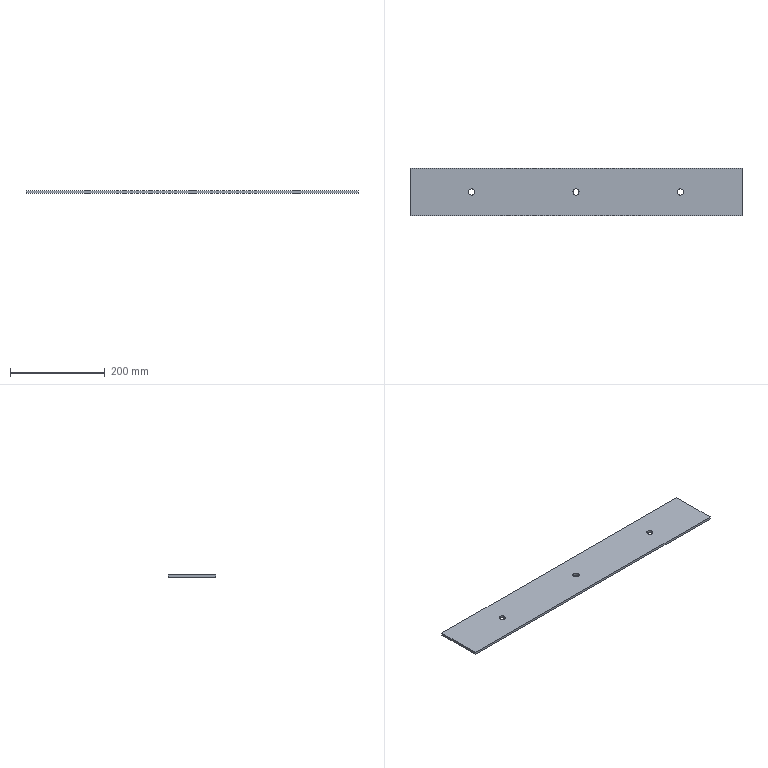Component | NX | SIDE_CONN_PLATE | 1 solid | 9 faces | box 700 x 100 x 5 mm | volume 348009 mm3 | plane 6 | cylinder 3 | commonest cylinder face diameters 13 x3
STEP:
#1=CARTESIAN_POINT('',(0.,0.,0.));
#2=DIRECTION('',(0.,0.,1.));
#3=DIRECTION('',(1.,0.,0.));
#4=AXIS2_PLACEMENT_3D('',#1,#2,#3);
#5=CARTESIAN_POINT('',(650.,50.,-525.));
#6=VERTEX_POINT('',#5);
#7=CARTESIAN_POINT('',(-50.,50.,-525.));
#8=VERTEX_POINT('',#7);
#9=CARTESIAN_POINT('',(650.,50.,-525.));
#10=DIRECTION('',(-1.,0.,0.));
#11=VECTOR('',#10,1.);
#12=LINE('',#9,#11);
#13=CARTESIAN_POINT('',(650.,50.,-530.));
#14=DIRECTION('',(0.,1.,0.));
#15=DIRECTION('',(0.,0.,1.));
#16=AXIS2_PLACEMENT_3D('',#13,#14,#15);
#17=PLANE('',#16);
#18=CARTESIAN_POINT('',(5.,0.));
#19=DIRECTION('',(0.,-1.));
#20=VECTOR('',#19,1.);
#21=LINE('',#18,#20);
#22=(GEOMETRIC_REPRESENTATION_CONTEXT(2)PARAMETRIC_REPRESENTATION_CONTEXT()REPRESENTATION_CONTEXT('',''));
#23=DEFINITIONAL_REPRESENTATION('',(#21),#22);
#24=PCURVE('',#17,#23);
#25=CARTESIAN_POINT('',(520.,-0.,-525.));
#26=DIRECTION('',(0.,0.,-1.));
#27=DIRECTION('',(1.,0.,0.));
#28=AXIS2_PLACEMENT_3D('',#25,#26,#27);
#29=PLANE('',#28);
#30=CARTESIAN_POINT('',(130.,-50.));
#31=DIRECTION('',(-1.,0.));
#32=VECTOR('',#31,1.);
#33=LINE('',#30,#32);
#34=(GEOMETRIC_REPRESENTATION_CONTEXT(2)PARAMETRIC_REPRESENTATION_CONTEXT()REPRESENTATION_CONTEXT('',''));
#35=DEFINITIONAL_REPRESENTATION('',(#33),#34);
#36=PCURVE('',#29,#35);
#37=SURFACE_CURVE('',#12,(#24,#36),.PCURVE_S1.);
#38=EDGE_CURVE('',#6,#8,#37,.T.);
#39=ORIENTED_EDGE('',*,*,#38,.F.);
#40=CARTESIAN_POINT('',(650.,50.,-530.));
#41=VERTEX_POINT('',#40);
#42=CARTESIAN_POINT('',(650.,50.,-530.));
#43=DIRECTION('',(0.,0.,1.));
#44=VECTOR('',#43,1.);
#45=LINE('',#42,#44);
#46=CARTESIAN_POINT('',(0.,0.));
#47=DIRECTION('',(1.,0.));
#48=VECTOR('',#47,1.);
#49=LINE('',#46,#48);
#50=(GEOMETRIC_REPRESENTATION_CONTEXT(2)PARAMETRIC_REPRESENTATION_CONTEXT()REPRESENTATION_CONTEXT('',''));
#51=DEFINITIONAL_REPRESENTATION('',(#49),#50);
#52=PCURVE('',#17,#51);
#53=CARTESIAN_POINT('',(650.,-50.,-530.));
#54=DIRECTION('',(1.,0.,0.));
#55=DIRECTION('',(0.,0.,1.));
#56=AXIS2_PLACEMENT_3D('',#53,#54,#55);
#57=PLANE('',#56);
#58=CARTESIAN_POINT('',(0.,-100.));
#59=DIRECTION('',(1.,0.));
#60=VECTOR('',#59,1.);
#61=LINE('',#58,#60);
#62=(GEOMETRIC_REPRESENTATION_CONTEXT(2)PARAMETRIC_REPRESENTATION_CONTEXT()REPRESENTATION_CONTEXT('',''));
#63=DEFINITIONAL_REPRESENTATION('',(#61),#62);
#64=PCURVE('',#57,#63);
#65=SURFACE_CURVE('',#45,(#52,#64),.PCURVE_S1.);
#66=EDGE_CURVE('',#41,#6,#65,.T.);
#67=ORIENTED_EDGE('',*,*,#66,.F.);
#68=CARTESIAN_POINT('',(-50.,50.,-530.));
#69=VERTEX_POINT('',#68);
#70=CARTESIAN_POINT('',(650.,50.,-530.));
#71=DIRECTION('',(-1.,0.,0.));
#72=VECTOR('',#71,1.);
#73=LINE('',#70,#72);
#74=CARTESIAN_POINT('',(0.,0.));
#75=DIRECTION('',(0.,-1.));
#76=VECTOR('',#75,1.);
#77=LINE('',#74,#76);
#78=(GEOMETRIC_REPRESENTATION_CONTEXT(2)PARAMETRIC_REPRESENTATION_CONTEXT()REPRESENTATION_CONTEXT('',''));
#79=DEFINITIONAL_REPRESENTATION('',(#77),#78);
#80=PCURVE('',#17,#79);
#81=CARTESIAN_POINT('',(520.,-0.,-530.));
#82=DIRECTION('',(0.,0.,-1.));
#83=DIRECTION('',(1.,0.,0.));
#84=AXIS2_PLACEMENT_3D('',#81,#82,#83);
#85=PLANE('',#84);
#86=CARTESIAN_POINT('',(130.,-50.));
#87=DIRECTION('',(-1.,0.));
#88=VECTOR('',#87,1.);
#89=LINE('',#86,#88);
#90=(GEOMETRIC_REPRESENTATION_CONTEXT(2)PARAMETRIC_REPRESENTATION_CONTEXT()REPRESENTATION_CONTEXT('',''));
#91=DEFINITIONAL_REPRESENTATION('',(#89),#90);
#92=PCURVE('',#85,#91);
#93=SURFACE_CURVE('',#73,(#80,#92),.PCURVE_S1.);
#94=EDGE_CURVE('',#41,#69,#93,.T.);
#95=ORIENTED_EDGE('',*,*,#94,.T.);
#96=CARTESIAN_POINT('',(-50.,50.,-530.));
#97=DIRECTION('',(0.,0.,1.));
#98=VECTOR('',#97,1.);
#99=LINE('',#96,#98);
#100=CARTESIAN_POINT('',(0.,-700.));
#101=DIRECTION('',(1.,0.));
#102=VECTOR('',#101,1.);
#103=LINE('',#100,#102);
#104=(GEOMETRIC_REPRESENTATION_CONTEXT(2)PARAMETRIC_REPRESENTATION_CONTEXT()REPRESENTATION_CONTEXT('',''));
#105=DEFINITIONAL_REPRESENTATION('',(#103),#104);
#106=PCURVE('',#17,#105);
#107=CARTESIAN_POINT('',(-50.,50.,-530.));
#108=DIRECTION('',(-1.,0.,0.));
#109=DIRECTION('',(0.,0.,-1.));
#110=AXIS2_PLACEMENT_3D('',#107,#108,#109);
#111=PLANE('',#110);
#112=CARTESIAN_POINT('',(0.,0.));
#113=DIRECTION('',(-1.,0.));
#114=VECTOR('',#113,1.);
#115=LINE('',#112,#114);
#116=(GEOMETRIC_REPRESENTATION_CONTEXT(2)PARAMETRIC_REPRESENTATION_CONTEXT()REPRESENTATION_CONTEXT('',''));
#117=DEFINITIONAL_REPRESENTATION('',(#115),#116);
#118=PCURVE('',#111,#117);
#119=SURFACE_CURVE('',#99,(#106,#118),.PCURVE_S1.);
#120=EDGE_CURVE('',#69,#8,#119,.T.);
#121=ORIENTED_EDGE('',*,*,#120,.T.);
#122=EDGE_LOOP('',(#39,#67,#95,#121));
#123=FACE_BOUND('',#122,.T.);
#124=ADVANCED_FACE('',(#123),#17,.T.);
#125=CARTESIAN_POINT('',(-50.,-50.,-525.));
#126=VERTEX_POINT('',#125);
#127=CARTESIAN_POINT('',(-50.,50.,-525.));
#128=DIRECTION('',(0.,-1.,0.));
#129=VECTOR('',#128,1.);
#130=LINE('',#127,#129);
#131=CARTESIAN_POINT('',(-5.,0.));
#132=DIRECTION('',(0.,1.));
#133=VECTOR('',#132,1.);
#134=LINE('',#131,#133);
#135=(GEOMETRIC_REPRESENTATION_CONTEXT(2)PARAMETRIC_REPRESENTATION_CONTEXT()REPRESENTATION_CONTEXT('',''));
#136=DEFINITIONAL_REPRESENTATION('',(#134),#135);
#137=PCURVE('',#111,#136);
#138=CARTESIAN_POINT('',(-570.,-50.));
#139=DIRECTION('',(0.,1.));
#140=VECTOR('',#139,1.);
#141=LINE('',#138,#140);
#142=(GEOMETRIC_REPRESENTATION_CONTEXT(2)PARAMETRIC_REPRESENTATION_CONTEXT()REPRESENTATION_CONTEXT('',''));
#143=DEFINITIONAL_REPRESENTATION('',(#141),#142);
#144=PCURVE('',#29,#143);
#145=SURFACE_CURVE('',#130,(#137,#144),.PCURVE_S1.);
#146=EDGE_CURVE('',#8,#126,#145,.T.);
#147=ORIENTED_EDGE('',*,*,#146,.F.);
#148=ORIENTED_EDGE('',*,*,#120,.F.);
#149=CARTESIAN_POINT('',(-50.,-50.,-530.));
#150=VERTEX_POINT('',#149);
#151=CARTESIAN_POINT('',(-50.,50.,-530.));
#152=DIRECTION('',(0.,-1.,0.));
#153=VECTOR('',#152,1.);
#154=LINE('',#151,#153);
#155=CARTESIAN_POINT('',(0.,0.));
#156=DIRECTION('',(0.,1.));
#157=VECTOR('',#156,1.);
#158=LINE('',#155,#157);
#159=(GEOMETRIC_REPRESENTATION_CONTEXT(2)PARAMETRIC_REPRESENTATION_CONTEXT()REPRESENTATION_CONTEXT('',''));
#160=DEFINITIONAL_REPRESENTATION('',(#158),#159);
#161=PCURVE('',#111,#160);
#162=CARTESIAN_POINT('',(-570.,-50.));
#163=DIRECTION('',(0.,1.));
#164=VECTOR('',#163,1.);
#165=LINE('',#162,#164);
#166=(GEOMETRIC_REPRESENTATION_CONTEXT(2)PARAMETRIC_REPRESENTATION_CONTEXT()REPRESENTATION_CONTEXT('',''));
#167=DEFINITIONAL_REPRESENTATION('',(#165),#166);
#168=PCURVE('',#85,#167);
#169=SURFACE_CURVE('',#154,(#161,#168),.PCURVE_S1.);
#170=EDGE_CURVE('',#69,#150,#169,.T.);
#171=ORIENTED_EDGE('',*,*,#170,.T.);
#172=CARTESIAN_POINT('',(-50.,-50.,-530.));
#173=DIRECTION('',(0.,0.,1.));
#174=VECTOR('',#173,1.);
#175=LINE('',#172,#174);
#176=CARTESIAN_POINT('',(0.,100.));
#177=DIRECTION('',(-1.,0.));
#178=VECTOR('',#177,1.);
#179=LINE('',#176,#178);
#180=(GEOMETRIC_REPRESENTATION_CONTEXT(2)PARAMETRIC_REPRESENTATION_CONTEXT()REPRESENTATION_CONTEXT('',''));
#181=DEFINITIONAL_REPRESENTATION('',(#179),#180);
#182=PCURVE('',#111,#181);
#183=CARTESIAN_POINT('',(-50.,-50.,-530.));
#184=DIRECTION('',(0.,-1.,0.));
#185=DIRECTION('',(0.,0.,-1.));
#186=AXIS2_PLACEMENT_3D('',#183,#184,#185);
#187=PLANE('',#186);
#188=CARTESIAN_POINT('',(0.,0.));
#189=DIRECTION('',(-1.,0.));
#190=VECTOR('',#189,1.);
#191=LINE('',#188,#190);
#192=(GEOMETRIC_REPRESENTATION_CONTEXT(2)PARAMETRIC_REPRESENTATION_CONTEXT()REPRESENTATION_CONTEXT('',''));
#193=DEFINITIONAL_REPRESENTATION('',(#191),#192);
#194=PCURVE('',#187,#193);
#195=SURFACE_CURVE('',#175,(#182,#194),.PCURVE_S1.);
#196=EDGE_CURVE('',#150,#126,#195,.T.);
#197=ORIENTED_EDGE('',*,*,#196,.T.);
#198=EDGE_LOOP('',(#147,#148,#171,#197));
#199=FACE_BOUND('',#198,.T.);
#200=ADVANCED_FACE('',(#199),#111,.T.);
#201=CARTESIAN_POINT('',(650.,-50.,-525.));
#202=VERTEX_POINT('',#201);
#203=CARTESIAN_POINT('',(-50.,-50.,-525.));
#204=DIRECTION('',(1.,0.,0.));
#205=VECTOR('',#204,1.);
#206=LINE('',#203,#205);
#207=CARTESIAN_POINT('',(-5.,0.));
#208=DIRECTION('',(0.,1.));
#209=VECTOR('',#208,1.);
#210=LINE('',#207,#209);
#211=(GEOMETRIC_REPRESENTATION_CONTEXT(2)PARAMETRIC_REPRESENTATION_CONTEXT()REPRESENTATION_CONTEXT('',''));
#212=DEFINITIONAL_REPRESENTATION('',(#210),#211);
#213=PCURVE('',#187,#212);
#214=CARTESIAN_POINT('',(-570.,50.));
#215=DIRECTION('',(1.,0.));
#216=VECTOR('',#215,1.);
#217=LINE('',#214,#216);
#218=(GEOMETRIC_REPRESENTATION_CONTEXT(2)PARAMETRIC_REPRESENTATION_CONTEXT()REPRESENTATION_CONTEXT('',''));
#219=DEFINITIONAL_REPRESENTATION('',(#217),#218);
#220=PCURVE('',#29,#219);
#221=SURFACE_CURVE('',#206,(#213,#220),.PCURVE_S1.);
#222=EDGE_CURVE('',#126,#202,#221,.T.);
#223=ORIENTED_EDGE('',*,*,#222,.F.);
#224=ORIENTED_EDGE('',*,*,#196,.F.);
#225=CARTESIAN_POINT('',(650.,-50.,-530.));
#226=VERTEX_POINT('',#225);
#227=CARTESIAN_POINT('',(-50.,-50.,-530.));
#228=DIRECTION('',(1.,0.,0.));
#229=VECTOR('',#228,1.);
#230=LINE('',#227,#229);
#231=CARTESIAN_POINT('',(0.,0.));
#232=DIRECTION('',(0.,1.));
#233=VECTOR('',#232,1.);
#234=LINE('',#231,#233);
#235=(GEOMETRIC_REPRESENTATION_CONTEXT(2)PARAMETRIC_REPRESENTATION_CONTEXT()REPRESENTATION_CONTEXT('',''));
#236=DEFINITIONAL_REPRESENTATION('',(#234),#235);
#237=PCURVE('',#187,#236);
#238=CARTESIAN_POINT('',(-570.,50.));
#239=DIRECTION('',(1.,0.));
#240=VECTOR('',#239,1.);
#241=LINE('',#238,#240);
#242=(GEOMETRIC_REPRESENTATION_CONTEXT(2)PARAMETRIC_REPRESENTATION_CONTEXT()REPRESENTATION_CONTEXT('',''));
#243=DEFINITIONAL_REPRESENTATION('',(#241),#242);
#244=PCURVE('',#85,#243);
#245=SURFACE_CURVE('',#230,(#237,#244),.PCURVE_S1.);
#246=EDGE_CURVE('',#150,#226,#245,.T.);
#247=ORIENTED_EDGE('',*,*,#246,.T.);
#248=CARTESIAN_POINT('',(650.,-50.,-530.));
#249=DIRECTION('',(0.,0.,1.));
#250=VECTOR('',#249,1.);
#251=LINE('',#248,#250);
#252=CARTESIAN_POINT('',(0.,700.));
#253=DIRECTION('',(-1.,0.));
#254=VECTOR('',#253,1.);
#255=LINE('',#252,#254);
#256=(GEOMETRIC_REPRESENTATION_CONTEXT(2)PARAMETRIC_REPRESENTATION_CONTEXT()REPRESENTATION_CONTEXT('',''));
#257=DEFINITIONAL_REPRESENTATION('',(#255),#256);
#258=PCURVE('',#187,#257);
#259=CARTESIAN_POINT('',(0.,0.));
#260=DIRECTION('',(1.,0.));
#261=VECTOR('',#260,1.);
#262=LINE('',#259,#261);
#263=(GEOMETRIC_REPRESENTATION_CONTEXT(2)PARAMETRIC_REPRESENTATION_CONTEXT()REPRESENTATION_CONTEXT('',''));
#264=DEFINITIONAL_REPRESENTATION('',(#262),#263);
#265=PCURVE('',#57,#264);
#266=SURFACE_CURVE('',#251,(#258,#265),.PCURVE_S1.);
#267=EDGE_CURVE('',#226,#202,#266,.T.);
#268=ORIENTED_EDGE('',*,*,#267,.T.);
#269=EDGE_LOOP('',(#223,#224,#247,#268));
#270=FACE_BOUND('',#269,.T.);
#271=ADVANCED_FACE('',(#270),#187,.T.);
#272=CARTESIAN_POINT('',(86.5,-0.,-530.));
#273=VERTEX_POINT('',#272);
#274=CARTESIAN_POINT('',(80.,-0.,-530.));
#275=DIRECTION('',(0.,0.,1.));
#276=DIRECTION('',(1.,-0.,0.));
#277=AXIS2_PLACEMENT_3D('',#274,#275,#276);
#278=CIRCLE('',#277,6.5);
#279=CARTESIAN_POINT('',(80.,-0.,-530.));
#280=DIRECTION('',(0.,0.,1.));
#281=DIRECTION('',(-1.,0.,0.));
#282=AXIS2_PLACEMENT_3D('',#279,#280,#281);
#283=CYLINDRICAL_SURFACE('',#282,6.5);
#284=CARTESIAN_POINT('',(3.142,0.));
#285=DIRECTION('',(1.,0.));
#286=VECTOR('',#285,1.);
#287=LINE('',#284,#286);
#288=(GEOMETRIC_REPRESENTATION_CONTEXT(2)PARAMETRIC_REPRESENTATION_CONTEXT()REPRESENTATION_CONTEXT('',''));
#289=DEFINITIONAL_REPRESENTATION('',(#287),#288);
#290=PCURVE('',#283,#289);
#291=CARTESIAN_POINT('',(-433.5,0.));
#292=CARTESIAN_POINT('',(-433.5,-11.258));
#293=CARTESIAN_POINT('',(-443.25,-5.629));
#294=CARTESIAN_POINT('',(-453.,-0.));
#295=CARTESIAN_POINT('',(-443.25,5.629));
#296=CARTESIAN_POINT('',(-433.5,11.258));
#297=CARTESIAN_POINT('',(-433.5,0.));
#298=(BOUNDED_CURVE()B_SPLINE_CURVE(2,(#291,#292,#293,#294,#295,#296,#297),.UNSPECIFIED.,.T.,.F.)B_SPLINE_CURVE_WITH_KNOTS((1,2,2,2,2,1),(-2.094,0.,2.094,4.189,6.283,8.378),.UNSPECIFIED.)CURVE()GEOMETRIC_REPRESENTATION_ITEM()RATIONAL_B_SPLINE_CURVE((1.,0.5,1.,0.5,1.,0.5,1.))REPRESENTATION_ITEM(''));
#299=(GEOMETRIC_REPRESENTATION_CONTEXT(2)PARAMETRIC_REPRESENTATION_CONTEXT()REPRESENTATION_CONTEXT('',''));
#300=DEFINITIONAL_REPRESENTATION('',(#298),#299);
#301=PCURVE('',#85,#300);
#302=SURFACE_CURVE('',#278,(#290,#301),.PCURVE_S1.);
#303=EDGE_CURVE('',#273,#273,#302,.T.);
#304=ORIENTED_EDGE('',*,*,#303,.T.);
#305=CARTESIAN_POINT('',(86.5,-0.,-525.));
#306=VERTEX_POINT('',#305);
#307=CARTESIAN_POINT('',(86.5,-0.,-530.));
#308=CARTESIAN_POINT('',(86.5,-0.,-525.));
#309=B_SPLINE_CURVE_WITH_KNOTS('',1,(#307,#308),.UNSPECIFIED.,.F.,.F.,(2,2),(0.,5.),.PIECEWISE_BEZIER_KNOTS.);
#310=CARTESIAN_POINT('',(9.425,0.));
#311=DIRECTION('',(0.,1.));
#312=VECTOR('',#311,1.);
#313=LINE('',#310,#312);
#314=(GEOMETRIC_REPRESENTATION_CONTEXT(2)PARAMETRIC_REPRESENTATION_CONTEXT()REPRESENTATION_CONTEXT('',''));
#315=DEFINITIONAL_REPRESENTATION('',(#313),#314);
#316=PCURVE('',#283,#315);
#317=CARTESIAN_POINT('',(3.142,0.));
#318=DIRECTION('',(0.,1.));
#319=VECTOR('',#318,1.);
#320=LINE('',#317,#319);
#321=(GEOMETRIC_REPRESENTATION_CONTEXT(2)PARAMETRIC_REPRESENTATION_CONTEXT()REPRESENTATION_CONTEXT('',''));
#322=DEFINITIONAL_REPRESENTATION('',(#320),#321);
#323=PCURVE('',#283,#322);
#324=SEAM_CURVE('',#309,(#316,#323),.PCURVE_S1.);
#325=EDGE_CURVE('',#273,#306,#324,.T.);
#326=ORIENTED_EDGE('',*,*,#325,.T.);
#327=CARTESIAN_POINT('',(80.,-0.,-525.));
#328=DIRECTION('',(0.,0.,1.));
#329=DIRECTION('',(1.,-0.,0.));
#330=AXIS2_PLACEMENT_3D('',#327,#328,#329);
#331=CIRCLE('',#330,6.5);
#332=CARTESIAN_POINT('',(3.142,5.));
#333=DIRECTION('',(1.,0.));
#334=VECTOR('',#333,1.);
#335=LINE('',#332,#334);
#336=(GEOMETRIC_REPRESENTATION_CONTEXT(2)PARAMETRIC_REPRESENTATION_CONTEXT()REPRESENTATION_CONTEXT('',''));
#337=DEFINITIONAL_REPRESENTATION('',(#335),#336);
#338=PCURVE('',#283,#337);
#339=CARTESIAN_POINT('',(-433.5,0.));
#340=CARTESIAN_POINT('',(-433.5,-11.258));
#341=CARTESIAN_POINT('',(-443.25,-5.629));
#342=CARTESIAN_POINT('',(-453.,-0.));
#343=CARTESIAN_POINT('',(-443.25,5.629));
#344=CARTESIAN_POINT('',(-433.5,11.258));
#345=CARTESIAN_POINT('',(-433.5,0.));
#346=(BOUNDED_CURVE()B_SPLINE_CURVE(2,(#339,#340,#341,#342,#343,#344,#345),.UNSPECIFIED.,.T.,.F.)B_SPLINE_CURVE_WITH_KNOTS((1,2,2,2,2,1),(-2.094,0.,2.094,4.189,6.283,8.378),.UNSPECIFIED.)CURVE()GEOMETRIC_REPRESENTATION_ITEM()RATIONAL_B_SPLINE_CURVE((1.,0.5,1.,0.5,1.,0.5,1.))REPRESENTATION_ITEM(''));
#347=(GEOMETRIC_REPRESENTATION_CONTEXT(2)PARAMETRIC_REPRESENTATION_CONTEXT()REPRESENTATION_CONTEXT('',''));
#348=DEFINITIONAL_REPRESENTATION('',(#346),#347);
#349=PCURVE('',#29,#348);
#350=SURFACE_CURVE('',#331,(#338,#349),.PCURVE_S1.);
#351=EDGE_CURVE('',#306,#306,#350,.T.);
#352=ORIENTED_EDGE('',*,*,#351,.F.);
#353=ORIENTED_EDGE('',*,*,#325,.F.);
#354=EDGE_LOOP('',(#304,#326,#352,#353));
#355=FACE_BOUND('',#354,.F.);
#356=ADVANCED_FACE('',(#355),#283,.F.);
#357=CARTESIAN_POINT('',(513.5,-0.,-530.));
#358=VERTEX_POINT('',#357);
#359=CARTESIAN_POINT('',(520.,-0.,-530.));
#360=DIRECTION('',(0.,0.,-1.));
#361=DIRECTION('',(-1.,-0.,0.));
#362=AXIS2_PLACEMENT_3D('',#359,#360,#361);
#363=CIRCLE('',#362,6.5);
#364=CARTESIAN_POINT('',(520.,-0.,-530.));
#365=DIRECTION('',(0.,0.,1.));
#366=DIRECTION('',(-1.,0.,0.));
#367=AXIS2_PLACEMENT_3D('',#364,#365,#366);
#368=CYLINDRICAL_SURFACE('',#367,6.5);
#369=CARTESIAN_POINT('',(6.283,0.));
#370=DIRECTION('',(-1.,0.));
#371=VECTOR('',#370,1.);
#372=LINE('',#369,#371);
#373=(GEOMETRIC_REPRESENTATION_CONTEXT(2)PARAMETRIC_REPRESENTATION_CONTEXT()REPRESENTATION_CONTEXT('',''));
#374=DEFINITIONAL_REPRESENTATION('',(#372),#373);
#375=PCURVE('',#368,#374);
#376=CARTESIAN_POINT('',(0.,0.));
#377=DIRECTION('',(-1.,0.));
#378=AXIS2_PLACEMENT_2D('',#376,#377);
#379=CIRCLE('',#378,6.5);
#380=(GEOMETRIC_REPRESENTATION_CONTEXT(2)PARAMETRIC_REPRESENTATION_CONTEXT()REPRESENTATION_CONTEXT('',''));
#381=DEFINITIONAL_REPRESENTATION('',(#379),#380);
#382=PCURVE('',#85,#381);
#383=SURFACE_CURVE('',#363,(#375,#382),.PCURVE_S1.);
#384=EDGE_CURVE('',#358,#358,#383,.T.);
#385=ORIENTED_EDGE('',*,*,#384,.F.);
#386=CARTESIAN_POINT('',(513.5,-0.,-525.));
#387=VERTEX_POINT('',#386);
#388=CARTESIAN_POINT('',(513.5,-0.,-530.));
#389=CARTESIAN_POINT('',(513.5,-0.,-525.));
#390=B_SPLINE_CURVE_WITH_KNOTS('',1,(#388,#389),.UNSPECIFIED.,.F.,.F.,(2,2),(0.,5.),.PIECEWISE_BEZIER_KNOTS.);
#391=CARTESIAN_POINT('',(6.283,0.));
#392=DIRECTION('',(0.,1.));
#393=VECTOR('',#392,1.);
#394=LINE('',#391,#393);
#395=(GEOMETRIC_REPRESENTATION_CONTEXT(2)PARAMETRIC_REPRESENTATION_CONTEXT()REPRESENTATION_CONTEXT('',''));
#396=DEFINITIONAL_REPRESENTATION('',(#394),#395);
#397=PCURVE('',#368,#396);
#398=CARTESIAN_POINT('',(0.,0.));
#399=DIRECTION('',(0.,1.));
#400=VECTOR('',#399,1.);
#401=LINE('',#398,#400);
#402=(GEOMETRIC_REPRESENTATION_CONTEXT(2)PARAMETRIC_REPRESENTATION_CONTEXT()REPRESENTATION_CONTEXT('',''));
#403=DEFINITIONAL_REPRESENTATION('',(#401),#402);
#404=PCURVE('',#368,#403);
#405=SEAM_CURVE('',#390,(#397,#404),.PCURVE_S1.);
#406=EDGE_CURVE('',#358,#387,#405,.T.);
#407=ORIENTED_EDGE('',*,*,#406,.T.);
#408=CARTESIAN_POINT('',(520.,-0.,-525.));
#409=DIRECTION('',(0.,0.,-1.));
#410=DIRECTION('',(-1.,-0.,0.));
#411=AXIS2_PLACEMENT_3D('',#408,#409,#410);
#412=CIRCLE('',#411,6.5);
#413=CARTESIAN_POINT('',(6.283,5.));
#414=DIRECTION('',(-1.,0.));
#415=VECTOR('',#414,1.);
#416=LINE('',#413,#415);
#417=(GEOMETRIC_REPRESENTATION_CONTEXT(2)PARAMETRIC_REPRESENTATION_CONTEXT()REPRESENTATION_CONTEXT('',''));
#418=DEFINITIONAL_REPRESENTATION('',(#416),#417);
#419=PCURVE('',#368,#418);
#420=CARTESIAN_POINT('',(0.,0.));
#421=DIRECTION('',(-1.,0.));
#422=AXIS2_PLACEMENT_2D('',#420,#421);
#423=CIRCLE('',#422,6.5);
#424=(GEOMETRIC_REPRESENTATION_CONTEXT(2)PARAMETRIC_REPRESENTATION_CONTEXT()REPRESENTATION_CONTEXT('',''));
#425=DEFINITIONAL_REPRESENTATION('',(#423),#424);
#426=PCURVE('',#29,#425);
#427=SURFACE_CURVE('',#412,(#419,#426),.PCURVE_S1.);
#428=EDGE_CURVE('',#387,#387,#427,.T.);
#429=ORIENTED_EDGE('',*,*,#428,.T.);
#430=ORIENTED_EDGE('',*,*,#406,.F.);
#431=EDGE_LOOP('',(#385,#407,#429,#430));
#432=FACE_BOUND('',#431,.F.);
#433=ADVANCED_FACE('',(#432),#368,.F.);
#434=CARTESIAN_POINT('',(650.,-50.,-525.));
#435=DIRECTION('',(0.,1.,0.));
#436=VECTOR('',#435,1.);
#437=LINE('',#434,#436);
#438=CARTESIAN_POINT('',(5.,0.));
#439=DIRECTION('',(0.,-1.));
#440=VECTOR('',#439,1.);
#441=LINE('',#438,#440);
#442=(GEOMETRIC_REPRESENTATION_CONTEXT(2)PARAMETRIC_REPRESENTATION_CONTEXT()REPRESENTATION_CONTEXT('',''));
#443=DEFINITIONAL_REPRESENTATION('',(#441),#442);
#444=PCURVE('',#57,#443);
#445=CARTESIAN_POINT('',(130.,50.));
#446=DIRECTION('',(0.,-1.));
#447=VECTOR('',#446,1.);
#448=LINE('',#445,#447);
#449=(GEOMETRIC_REPRESENTATION_CONTEXT(2)PARAMETRIC_REPRESENTATION_CONTEXT()REPRESENTATION_CONTEXT('',''));
#450=DEFINITIONAL_REPRESENTATION('',(#448),#449);
#451=PCURVE('',#29,#450);
#452=SURFACE_CURVE('',#437,(#444,#451),.PCURVE_S1.);
#453=EDGE_CURVE('',#202,#6,#452,.T.);
#454=ORIENTED_EDGE('',*,*,#453,.F.);
#455=ORIENTED_EDGE('',*,*,#267,.F.);
#456=CARTESIAN_POINT('',(650.,-50.,-530.));
#457=DIRECTION('',(0.,1.,0.));
#458=VECTOR('',#457,1.);
#459=LINE('',#456,#458);
#460=CARTESIAN_POINT('',(0.,0.));
#461=DIRECTION('',(0.,-1.));
#462=VECTOR('',#461,1.);
#463=LINE('',#460,#462);
#464=(GEOMETRIC_REPRESENTATION_CONTEXT(2)PARAMETRIC_REPRESENTATION_CONTEXT()REPRESENTATION_CONTEXT('',''));
#465=DEFINITIONAL_REPRESENTATION('',(#463),#464);
#466=PCURVE('',#57,#465);
#467=CARTESIAN_POINT('',(130.,50.));
#468=DIRECTION('',(0.,-1.));
#469=VECTOR('',#468,1.);
#470=LINE('',#467,#469);
#471=(GEOMETRIC_REPRESENTATION_CONTEXT(2)PARAMETRIC_REPRESENTATION_CONTEXT()REPRESENTATION_CONTEXT('',''));
#472=DEFINITIONAL_REPRESENTATION('',(#470),#471);
#473=PCURVE('',#85,#472);
#474=SURFACE_CURVE('',#459,(#466,#473),.PCURVE_S1.);
#475=EDGE_CURVE('',#226,#41,#474,.T.);
#476=ORIENTED_EDGE('',*,*,#475,.T.);
#477=ORIENTED_EDGE('',*,*,#66,.T.);
#478=EDGE_LOOP('',(#454,#455,#476,#477));
#479=FACE_BOUND('',#478,.T.);
#480=ADVANCED_FACE('',(#479),#57,.T.);
#481=CARTESIAN_POINT('',(306.5,-0.,-530.));
#482=VERTEX_POINT('',#481);
#483=CARTESIAN_POINT('',(300.,-0.,-530.));
#484=DIRECTION('',(0.,0.,1.));
#485=DIRECTION('',(1.,-0.,0.));
#486=AXIS2_PLACEMENT_3D('',#483,#484,#485);
#487=CIRCLE('',#486,6.5);
#488=CARTESIAN_POINT('',(300.,-0.,-530.));
#489=DIRECTION('',(0.,0.,1.));
#490=DIRECTION('',(-1.,0.,0.));
#491=AXIS2_PLACEMENT_3D('',#488,#489,#490);
#492=CYLINDRICAL_SURFACE('',#491,6.5);
#493=CARTESIAN_POINT('',(3.142,0.));
#494=DIRECTION('',(1.,0.));
#495=VECTOR('',#494,1.);
#496=LINE('',#493,#495);
#497=(GEOMETRIC_REPRESENTATION_CONTEXT(2)PARAMETRIC_REPRESENTATION_CONTEXT()REPRESENTATION_CONTEXT('',''));
#498=DEFINITIONAL_REPRESENTATION('',(#496),#497);
#499=PCURVE('',#492,#498);
#500=CARTESIAN_POINT('',(-213.5,0.));
#501=CARTESIAN_POINT('',(-213.5,-11.258));
#502=CARTESIAN_POINT('',(-223.25,-5.629));
#503=CARTESIAN_POINT('',(-233.,-0.));
#504=CARTESIAN_POINT('',(-223.25,5.629));
#505=CARTESIAN_POINT('',(-213.5,11.258));
#506=CARTESIAN_POINT('',(-213.5,0.));
#507=(BOUNDED_CURVE()B_SPLINE_CURVE(2,(#500,#501,#502,#503,#504,#505,#506),.UNSPECIFIED.,.T.,.F.)B_SPLINE_CURVE_WITH_KNOTS((1,2,2,2,2,1),(-2.094,0.,2.094,4.189,6.283,8.378),.UNSPECIFIED.)CURVE()GEOMETRIC_REPRESENTATION_ITEM()RATIONAL_B_SPLINE_CURVE((1.,0.5,1.,0.5,1.,0.5,1.))REPRESENTATION_ITEM(''));
#508=(GEOMETRIC_REPRESENTATION_CONTEXT(2)PARAMETRIC_REPRESENTATION_CONTEXT()REPRESENTATION_CONTEXT('',''));
#509=DEFINITIONAL_REPRESENTATION('',(#507),#508);
#510=PCURVE('',#85,#509);
#511=SURFACE_CURVE('',#487,(#499,#510),.PCURVE_S1.);
#512=EDGE_CURVE('',#482,#482,#511,.T.);
#513=ORIENTED_EDGE('',*,*,#512,.T.);
#514=CARTESIAN_POINT('',(306.5,-0.,-525.));
#515=VERTEX_POINT('',#514);
#516=CARTESIAN_POINT('',(306.5,-0.,-530.));
#517=CARTESIAN_POINT('',(306.5,-0.,-525.));
#518=B_SPLINE_CURVE_WITH_KNOTS('',1,(#516,#517),.UNSPECIFIED.,.F.,.F.,(2,2),(0.,5.),.PIECEWISE_BEZIER_KNOTS.);
#519=CARTESIAN_POINT('',(9.425,0.));
#520=DIRECTION('',(0.,1.));
#521=VECTOR('',#520,1.);
#522=LINE('',#519,#521);
#523=(GEOMETRIC_REPRESENTATION_CONTEXT(2)PARAMETRIC_REPRESENTATION_CONTEXT()REPRESENTATION_CONTEXT('',''));
#524=DEFINITIONAL_REPRESENTATION('',(#522),#523);
#525=PCURVE('',#492,#524);
#526=CARTESIAN_POINT('',(3.142,0.));
#527=DIRECTION('',(0.,1.));
#528=VECTOR('',#527,1.);
#529=LINE('',#526,#528);
#530=(GEOMETRIC_REPRESENTATION_CONTEXT(2)PARAMETRIC_REPRESENTATION_CONTEXT()REPRESENTATION_CONTEXT('',''));
#531=DEFINITIONAL_REPRESENTATION('',(#529),#530);
#532=PCURVE('',#492,#531);
#533=SEAM_CURVE('',#518,(#525,#532),.PCURVE_S1.);
#534=EDGE_CURVE('',#482,#515,#533,.T.);
#535=ORIENTED_EDGE('',*,*,#534,.T.);
#536=CARTESIAN_POINT('',(300.,-0.,-525.));
#537=DIRECTION('',(0.,0.,1.));
#538=DIRECTION('',(1.,-0.,0.));
#539=AXIS2_PLACEMENT_3D('',#536,#537,#538);
#540=CIRCLE('',#539,6.5);
#541=CARTESIAN_POINT('',(3.142,5.));
#542=DIRECTION('',(1.,0.));
#543=VECTOR('',#542,1.);
#544=LINE('',#541,#543);
#545=(GEOMETRIC_REPRESENTATION_CONTEXT(2)PARAMETRIC_REPRESENTATION_CONTEXT()REPRESENTATION_CONTEXT('',''));
#546=DEFINITIONAL_REPRESENTATION('',(#544),#545);
#547=PCURVE('',#492,#546);
#548=CARTESIAN_POINT('',(-213.5,0.));
#549=CARTESIAN_POINT('',(-213.5,-11.258));
#550=CARTESIAN_POINT('',(-223.25,-5.629));
#551=CARTESIAN_POINT('',(-233.,-0.));
#552=CARTESIAN_POINT('',(-223.25,5.629));
#553=CARTESIAN_POINT('',(-213.5,11.258));
#554=CARTESIAN_POINT('',(-213.5,0.));
#555=(BOUNDED_CURVE()B_SPLINE_CURVE(2,(#548,#549,#550,#551,#552,#553,#554),.UNSPECIFIED.,.T.,.F.)B_SPLINE_CURVE_WITH_KNOTS((1,2,2,2,2,1),(-2.094,0.,2.094,4.189,6.283,8.378),.UNSPECIFIED.)CURVE()GEOMETRIC_REPRESENTATION_ITEM()RATIONAL_B_SPLINE_CURVE((1.,0.5,1.,0.5,1.,0.5,1.))REPRESENTATION_ITEM(''));
#556=(GEOMETRIC_REPRESENTATION_CONTEXT(2)PARAMETRIC_REPRESENTATION_CONTEXT()REPRESENTATION_CONTEXT('',''));
#557=DEFINITIONAL_REPRESENTATION('',(#555),#556);
#558=PCURVE('',#29,#557);
#559=SURFACE_CURVE('',#540,(#547,#558),.PCURVE_S1.);
#560=EDGE_CURVE('',#515,#515,#559,.T.);
#561=ORIENTED_EDGE('',*,*,#560,.F.);
#562=ORIENTED_EDGE('',*,*,#534,.F.);
#563=EDGE_LOOP('',(#513,#535,#561,#562));
#564=FACE_BOUND('',#563,.F.);
#565=ADVANCED_FACE('',(#564),#492,.F.);
#566=ORIENTED_EDGE('',*,*,#94,.F.);
#567=ORIENTED_EDGE('',*,*,#475,.F.);
#568=ORIENTED_EDGE('',*,*,#246,.F.);
#569=ORIENTED_EDGE('',*,*,#170,.F.);
#570=EDGE_LOOP('',(#566,#567,#568,#569));
#571=FACE_BOUND('',#570,.T.);
#572=ORIENTED_EDGE('',*,*,#384,.F.);
#573=EDGE_LOOP('',(#572));
#574=FACE_BOUND('',#573,.T.);
#575=ORIENTED_EDGE('',*,*,#303,.T.);
#576=EDGE_LOOP('',(#575));
#577=FACE_BOUND('',#576,.T.);
#578=ORIENTED_EDGE('',*,*,#512,.T.);
#579=EDGE_LOOP('',(#578));
#580=FACE_BOUND('',#579,.T.);
#581=ADVANCED_FACE('',(#571,#574,#577,#580),#85,.T.);
#582=ORIENTED_EDGE('',*,*,#38,.T.);
#583=ORIENTED_EDGE('',*,*,#146,.T.);
#584=ORIENTED_EDGE('',*,*,#222,.T.);
#585=ORIENTED_EDGE('',*,*,#453,.T.);
#586=EDGE_LOOP('',(#582,#583,#584,#585));
#587=FACE_BOUND('',#586,.T.);
#588=ORIENTED_EDGE('',*,*,#428,.T.);
#589=EDGE_LOOP('',(#588));
#590=FACE_BOUND('',#589,.T.);
#591=ORIENTED_EDGE('',*,*,#351,.F.);
#592=EDGE_LOOP('',(#591));
#593=FACE_BOUND('',#592,.T.);
#594=ORIENTED_EDGE('',*,*,#560,.F.);
#595=EDGE_LOOP('',(#594));
#596=FACE_BOUND('',#595,.T.);
#597=ADVANCED_FACE('',(#587,#590,#593,#596),#29,.F.);
#598=CLOSED_SHELL('',(#124,#200,#271,#356,#433,#480,#565,#581,#597));
#599=MANIFOLD_SOLID_BREP('',#598);
#600=(LENGTH_UNIT()NAMED_UNIT(*)SI_UNIT(.MILLI.,.METRE.));
#601=UNCERTAINTY_MEASURE_WITH_UNIT(LENGTH_MEASURE(0.000002),#600,'','');
#602=(NAMED_UNIT(*)PLANE_ANGLE_UNIT()SI_UNIT($,.RADIAN.));
#603=(NAMED_UNIT(*)SI_UNIT($,.STERADIAN.)SOLID_ANGLE_UNIT());
#604=(GEOMETRIC_REPRESENTATION_CONTEXT(3)GLOBAL_UNCERTAINTY_ASSIGNED_CONTEXT((#601))GLOBAL_UNIT_ASSIGNED_CONTEXT((#600,#602,#603))REPRESENTATION_CONTEXT('',''));
#605=ADVANCED_BREP_SHAPE_REPRESENTATION('',(#4,#599),#604);